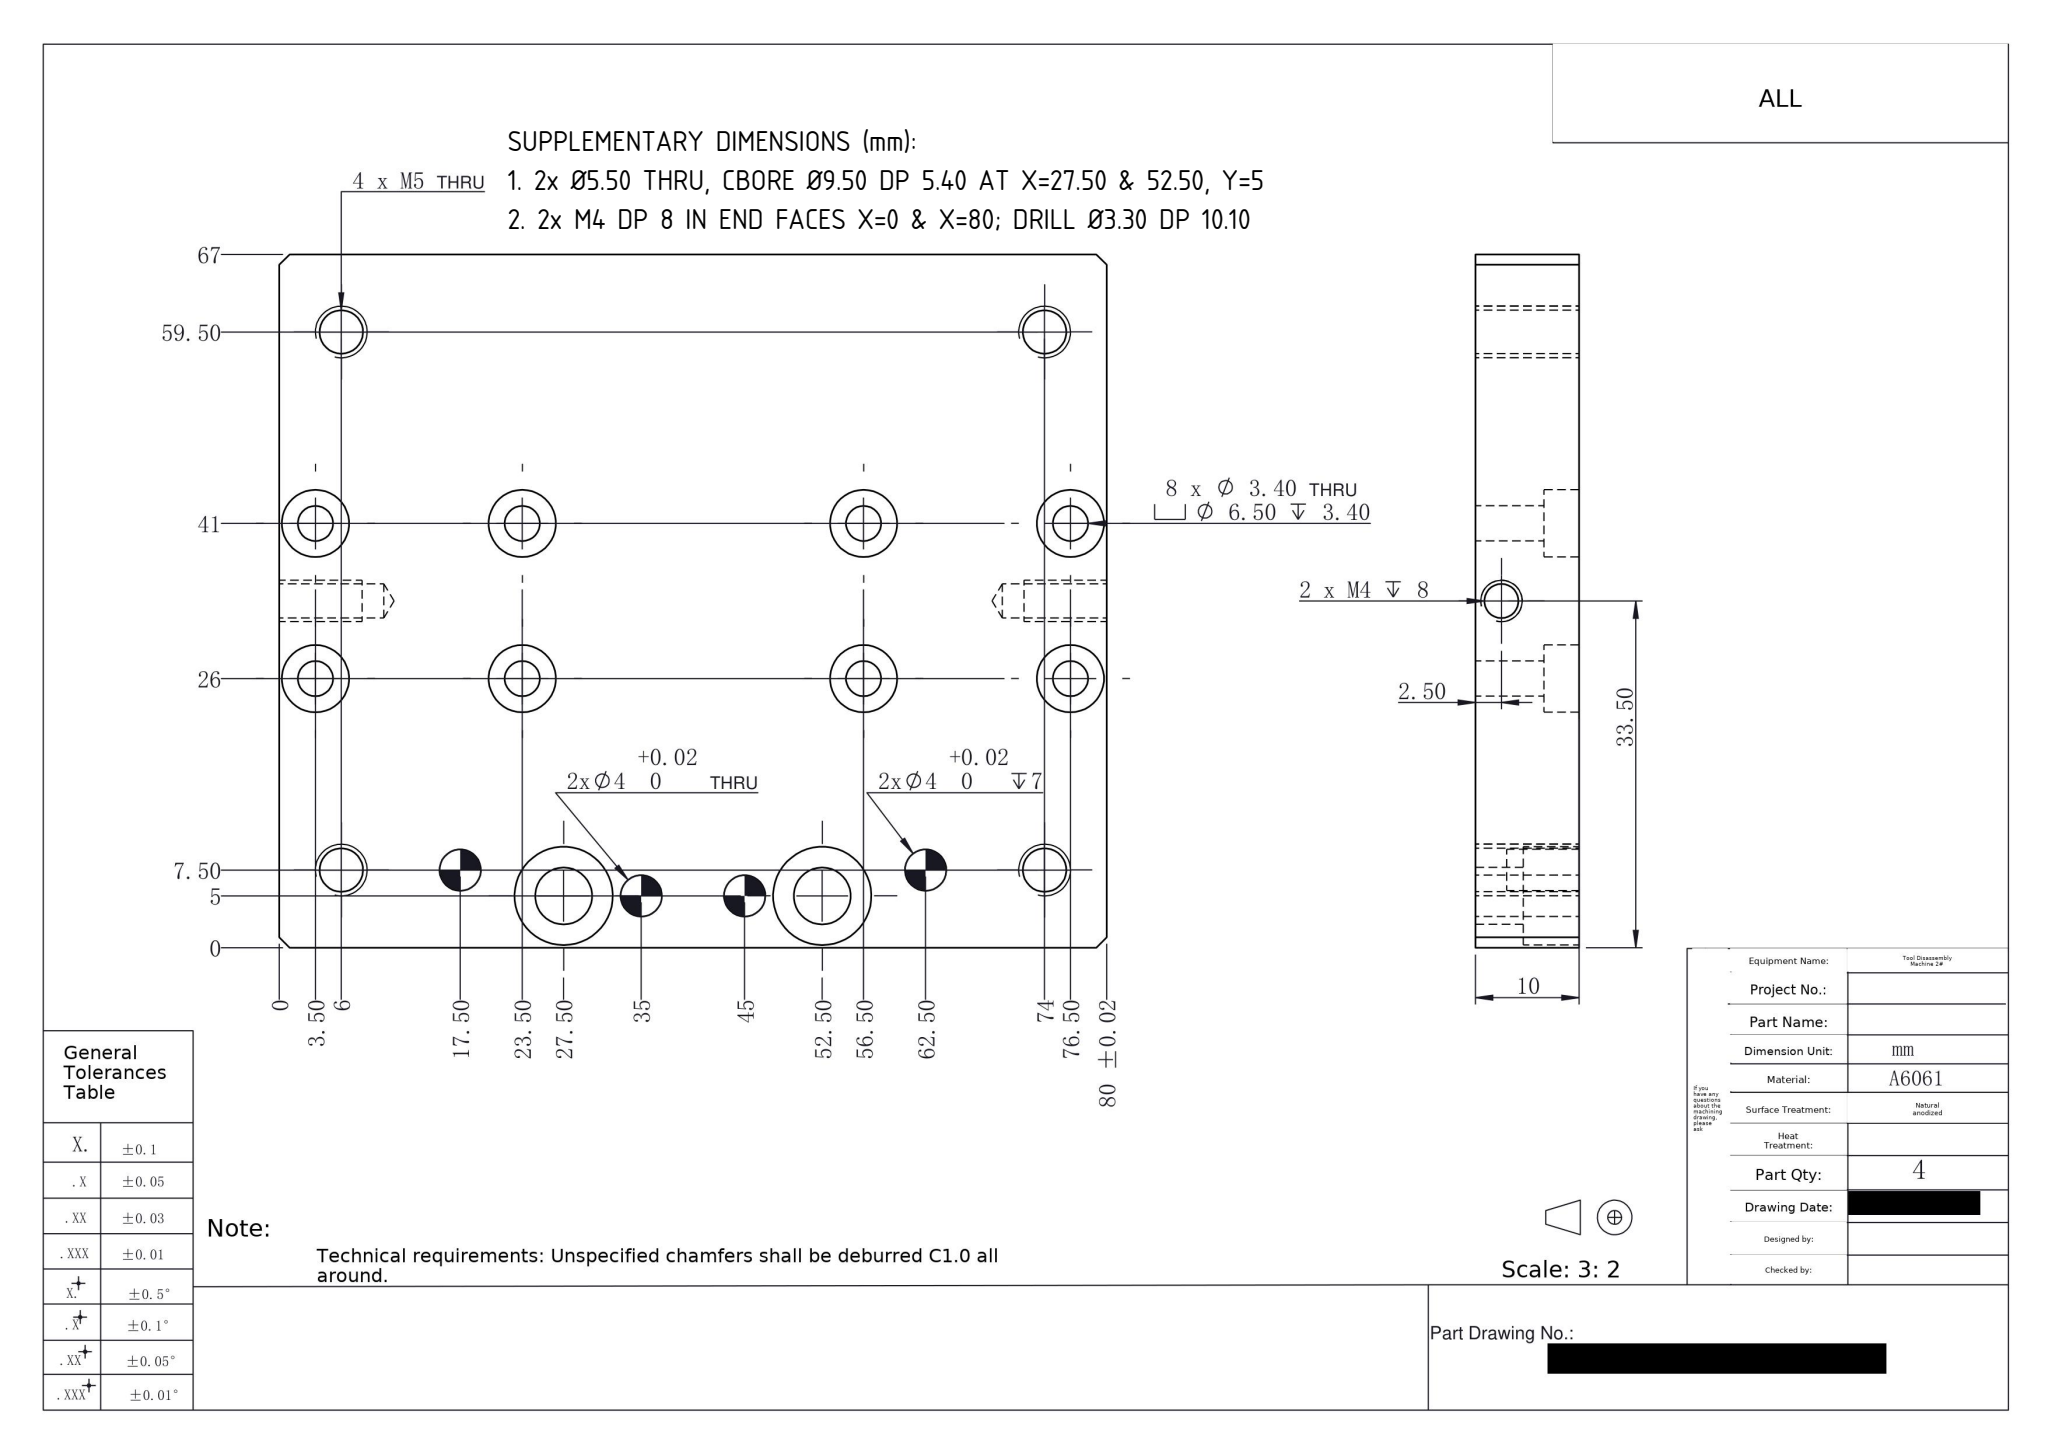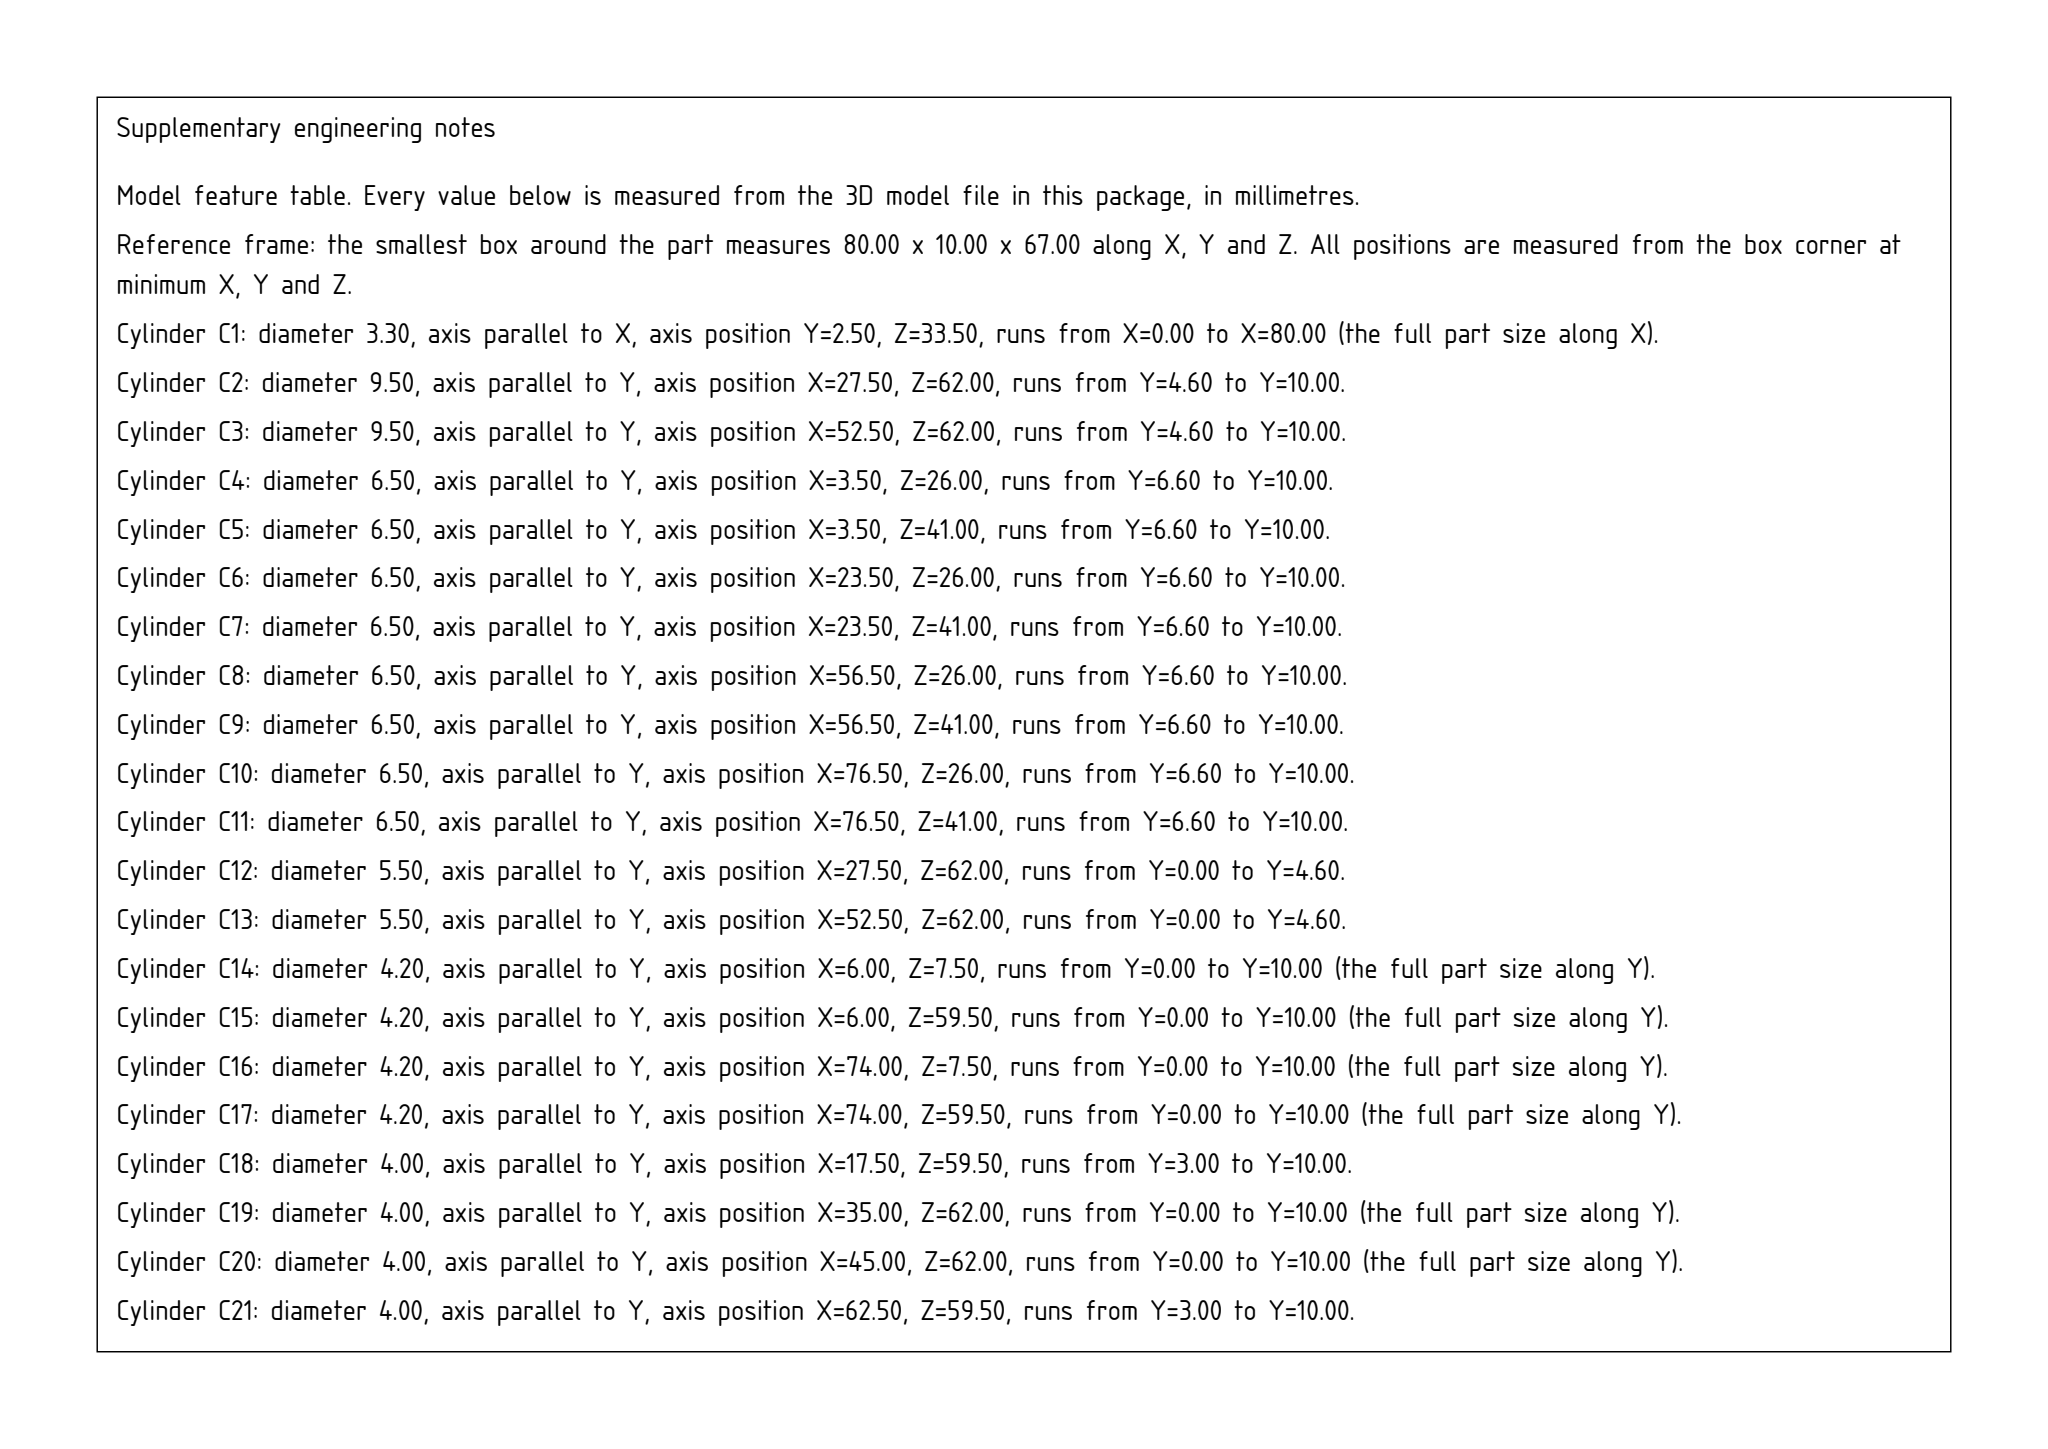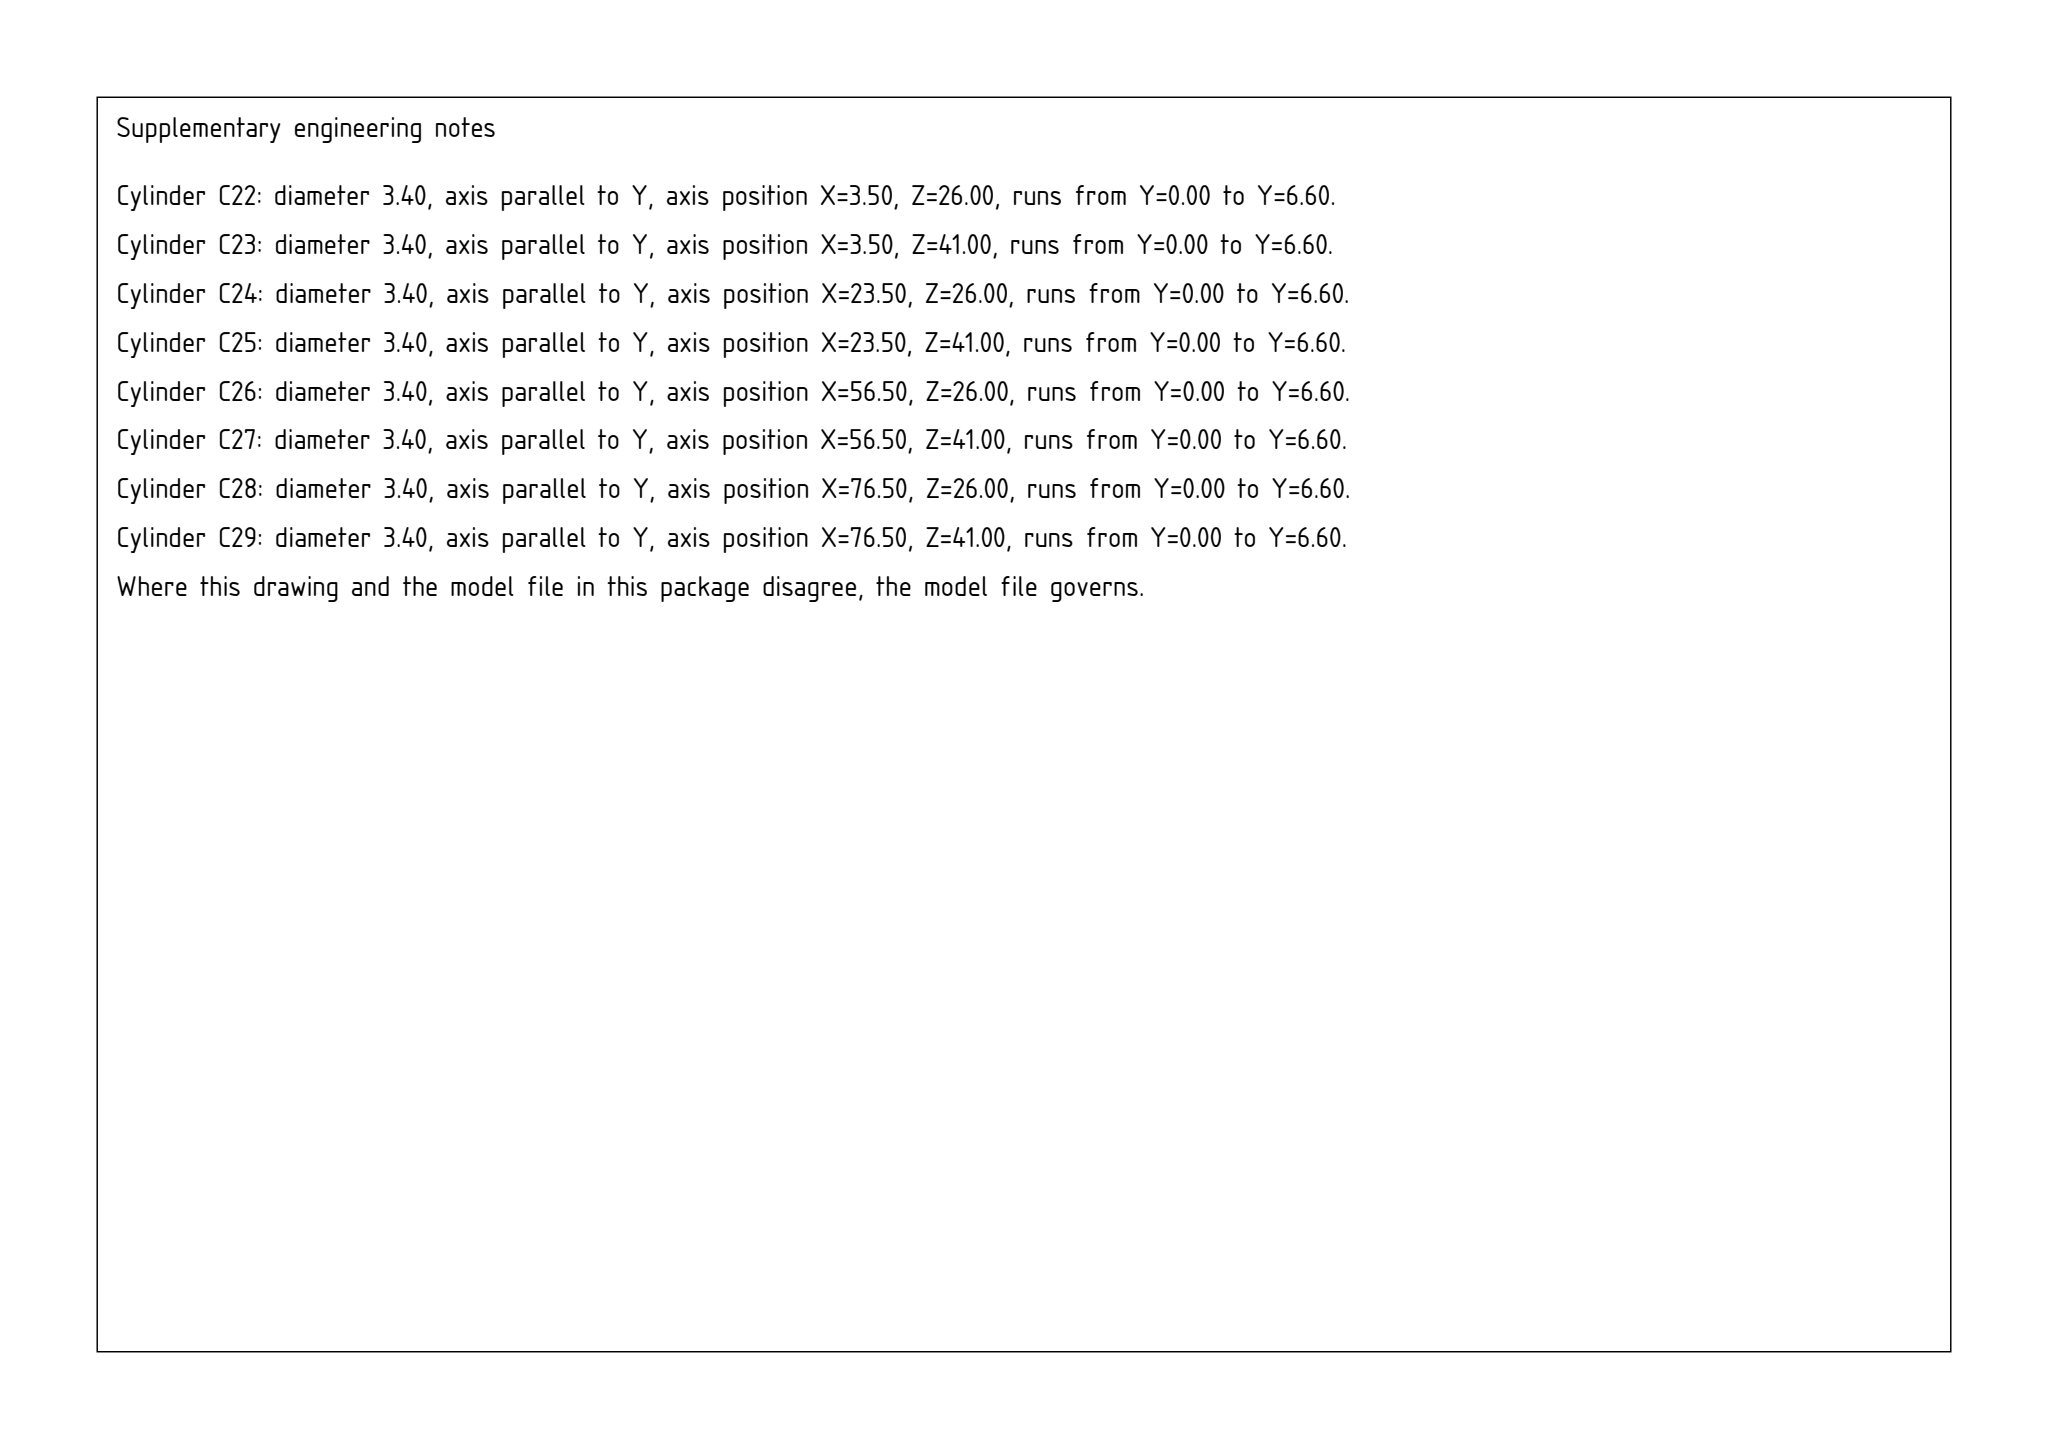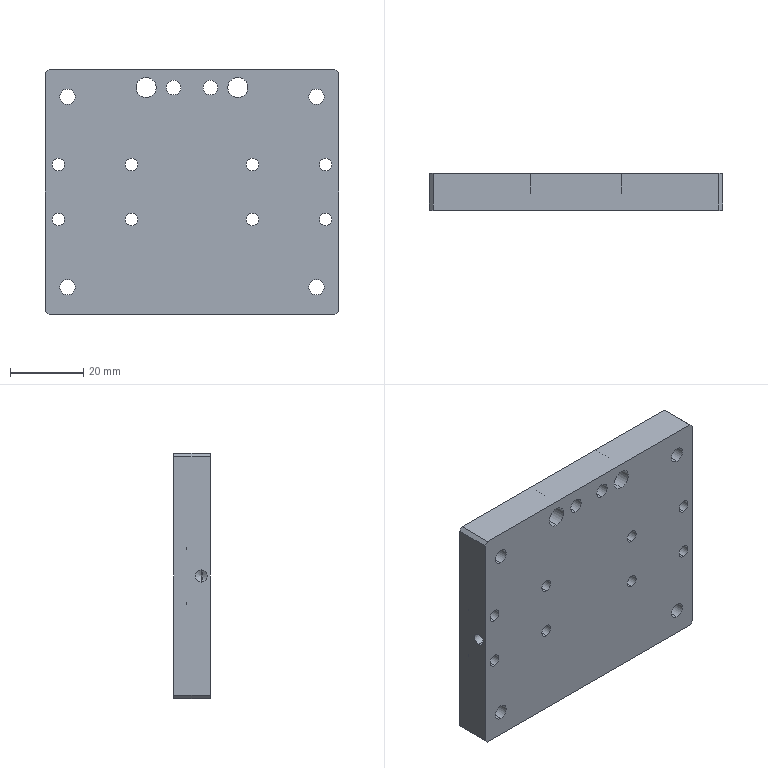Part | SolidWorks | mm | 1 solid | 86 faces | box 80 x 10 x 67 mm | volume 50054 mm3 | cylinder 60 | plane 22 | cone 4 | commonest cylinder face diameters 6.5 x16 3.4 x16 4 x8 4.2 x8 9.5 x4 5.5 x4 3.3 x4
build123d program:
from build123d import *

# Parameters (mm, degrees)
SKETCH1_W                                       = 80
SKETCH1_H                                       = 67
BOSS_EXTRUDE1_DEPTH                             = 5
M5_TAPPED_HOLE1_D                               = 4.2
M3_HEX_SOCKET_HEAD_CAP_SCREW_CBORE1_D           = 3.4
M3_HEX_SOCKET_HEAD_CAP_SCREW_CBORE1_CBORE_D     = 6.5
M3_HEX_SOCKET_HEAD_CAP_SCREW_CBORE1_CBORE_DEPTH = 3.4
M5_HEX_SOCKET_HEAD_CAP_SCREW_CBORE1_D           = 5.5
M5_HEX_SOCKET_HEAD_CAP_SCREW_CBORE1_CBORE_D     = 9.5
M5_HEX_SOCKET_HEAD_CAP_SCREW_CBORE1_CBORE_DEPTH = 5.4
F_4_0MM_DOWEL_PIN_HOLE1_D                       = 4
F_4_0MM_DOWEL_PIN_HOLE2_D                       = 4
F_4_0MM_DOWEL_PIN_HOLE2_DEPTH                   = 7
CHAMFER1_SIZE                                   = 1


with BuildPart() as part:
    # Sketch1 → Boss-Extrude1 (new, symmetric)
    with BuildSketch(Plane(origin=(0, 0, 0), x_dir=(1, 0, 0), z_dir=(0, 1, 0))):
        Rectangle(SKETCH1_W, SKETCH1_H)
    extrude(amount=BOSS_EXTRUDE1_DEPTH, both=True)

    # M5 Tapped Hole1 (through all)
    with Locations(Plane(origin=(0, 5, 0), x_dir=(1, 0, 0), z_dir=(0, 1, 0))):
        with Locations((-34, 26), (-34, -26), (34, -26), (34, 26)):
            Hole(M5_TAPPED_HOLE1_D / 2)

    # M3 Hex Socket Head Cap Screw CBORE1 (through all)
    with Locations(Plane(origin=(0, 5, 0), x_dir=(1, 0, 0), z_dir=(0, 1, 0))):
        with Locations((16.5, 7.5), (16.5, -7.5), (36.5, -7.5), (36.5, 7.5)):
            m3_hex_socket_head_cap_screw_cbore1 = CounterBoreHole(M3_HEX_SOCKET_HEAD_CAP_SCREW_CBORE1_D / 2, M3_HEX_SOCKET_HEAD_CAP_SCREW_CBORE1_CBORE_D / 2, M3_HEX_SOCKET_HEAD_CAP_SCREW_CBORE1_CBORE_DEPTH)

    # Sketch7 → M4 Tapped Hole1 (revolve, cut)
    with BuildSketch(Plane(origin=(40, -2.5, 0), x_dir=(0, 0, -1), z_dir=(0, 1, 0))):
        Polygon((0, 0), (0, 11.091), (1.65, 10.1), (1.65, 0), align=None)
    m4_tapped_hole1 = revolve(axis=Axis((46.35, -2.5, 0), (-1, 0, 0)), mode=Mode.SUBTRACT)

    # Mirror1: M3 Hex Socket Head Cap Screw CBORE1, M4 Tapped Hole1 across plane
    add(m3_hex_socket_head_cap_screw_cbore1.mirror(Plane(origin=(0, 0, 0), x_dir=(0, 0, 1), z_dir=(1, 0, 0))), mode=Mode.SUBTRACT)
    add(m4_tapped_hole1.mirror(Plane(origin=(0, 0, 0), x_dir=(0, 0, 1), z_dir=(1, 0, 0))), mode=Mode.SUBTRACT)

    # M5 Hex Socket Head Cap Screw CBORE1 (through all)
    with Locations(Plane(origin=(0, 5, 0), x_dir=(1, 0, 0), z_dir=(0, 1, 0))):
        with Locations((-12.5, -28.5), (12.5, -28.5)):
            CounterBoreHole(M5_HEX_SOCKET_HEAD_CAP_SCREW_CBORE1_D / 2, M5_HEX_SOCKET_HEAD_CAP_SCREW_CBORE1_CBORE_D / 2, M5_HEX_SOCKET_HEAD_CAP_SCREW_CBORE1_CBORE_DEPTH)

    # 4.0mm Dowel Pin Hole1 (through all)
    with Locations(Plane(origin=(0, 5, 0), x_dir=(1, 0, 0), z_dir=(0, 1, 0))):
        with Locations((-5, -28.5), (5, -28.5)):
            Hole(F_4_0MM_DOWEL_PIN_HOLE1_D / 2)

    # 4.0mm Dowel Pin Hole2
    with Locations(Plane(origin=(0, 5, 0), x_dir=(1, 0, 0), z_dir=(0, 1, 0))):
        with Locations((-22.5, -26), (22.5, -26)):
            Hole(F_4_0MM_DOWEL_PIN_HOLE2_D / 2, depth=F_4_0MM_DOWEL_PIN_HOLE2_DEPTH)

    # Chamfer1
    chamfer1_edges = [part.edges().sort_by_distance(p)[0] for p in [
        (40, 0, 33.5),
        (-40, 0, 33.5),
        (-40, 0, -33.5),
        (40, 0, -33.5),
    ]]
    chamfer(chamfer1_edges, length=CHAMFER1_SIZE)


solid = part.part